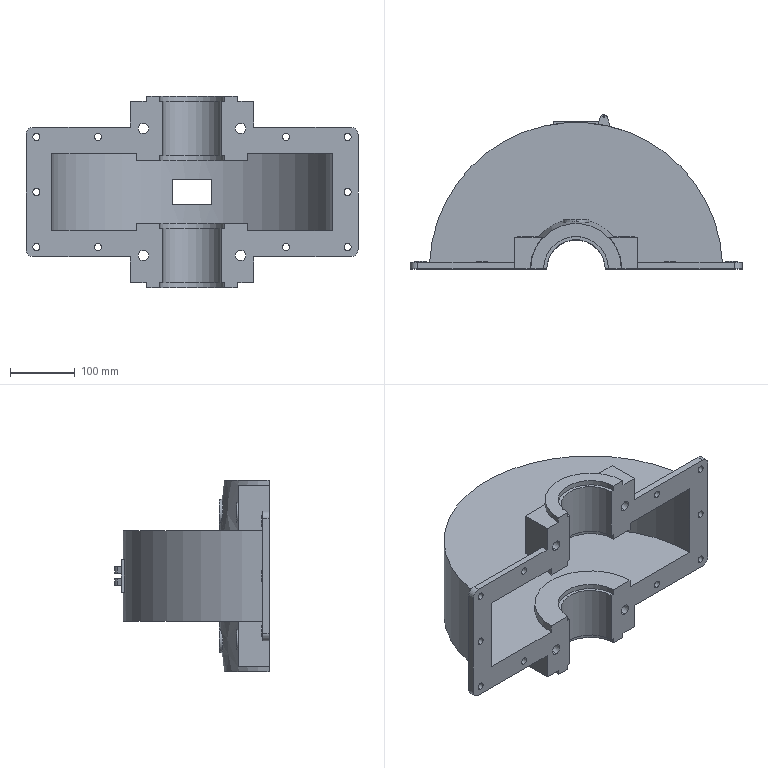Component | SolidWorks | 1CoverBox-1 | 1 solid | 163 faces | volume 3955776 mm3 | cylinder 84 | plane 69 | cone 10 | commonest cylinder face diameters 11 x20 18 x20 16 x8 30 x8 3 x4 17.5 x4 40 x4 24 x4